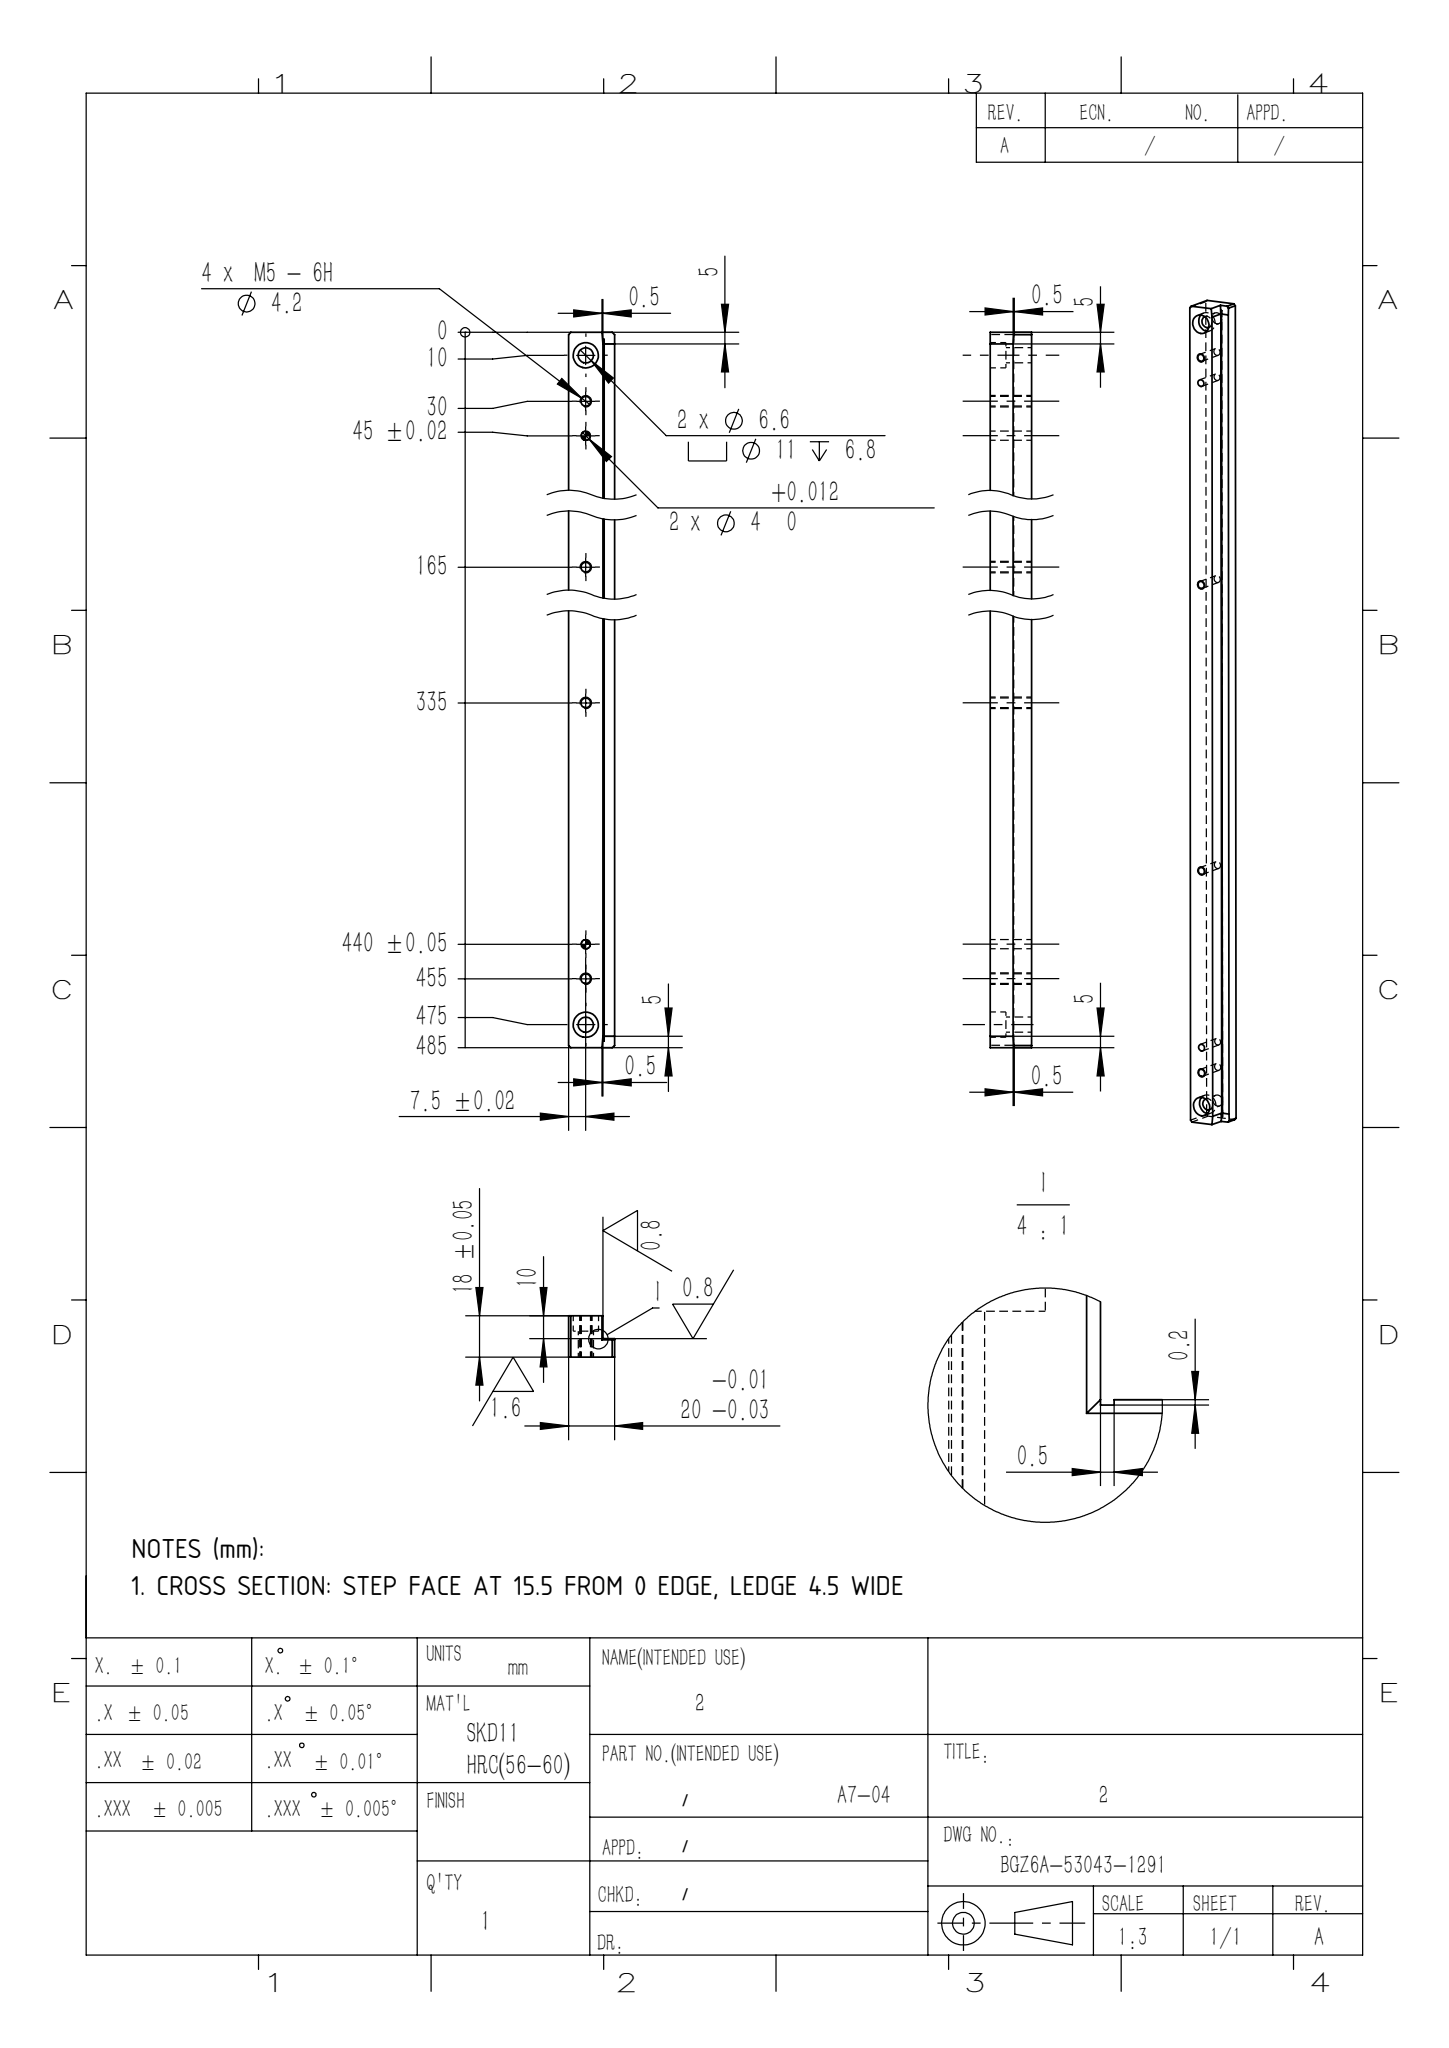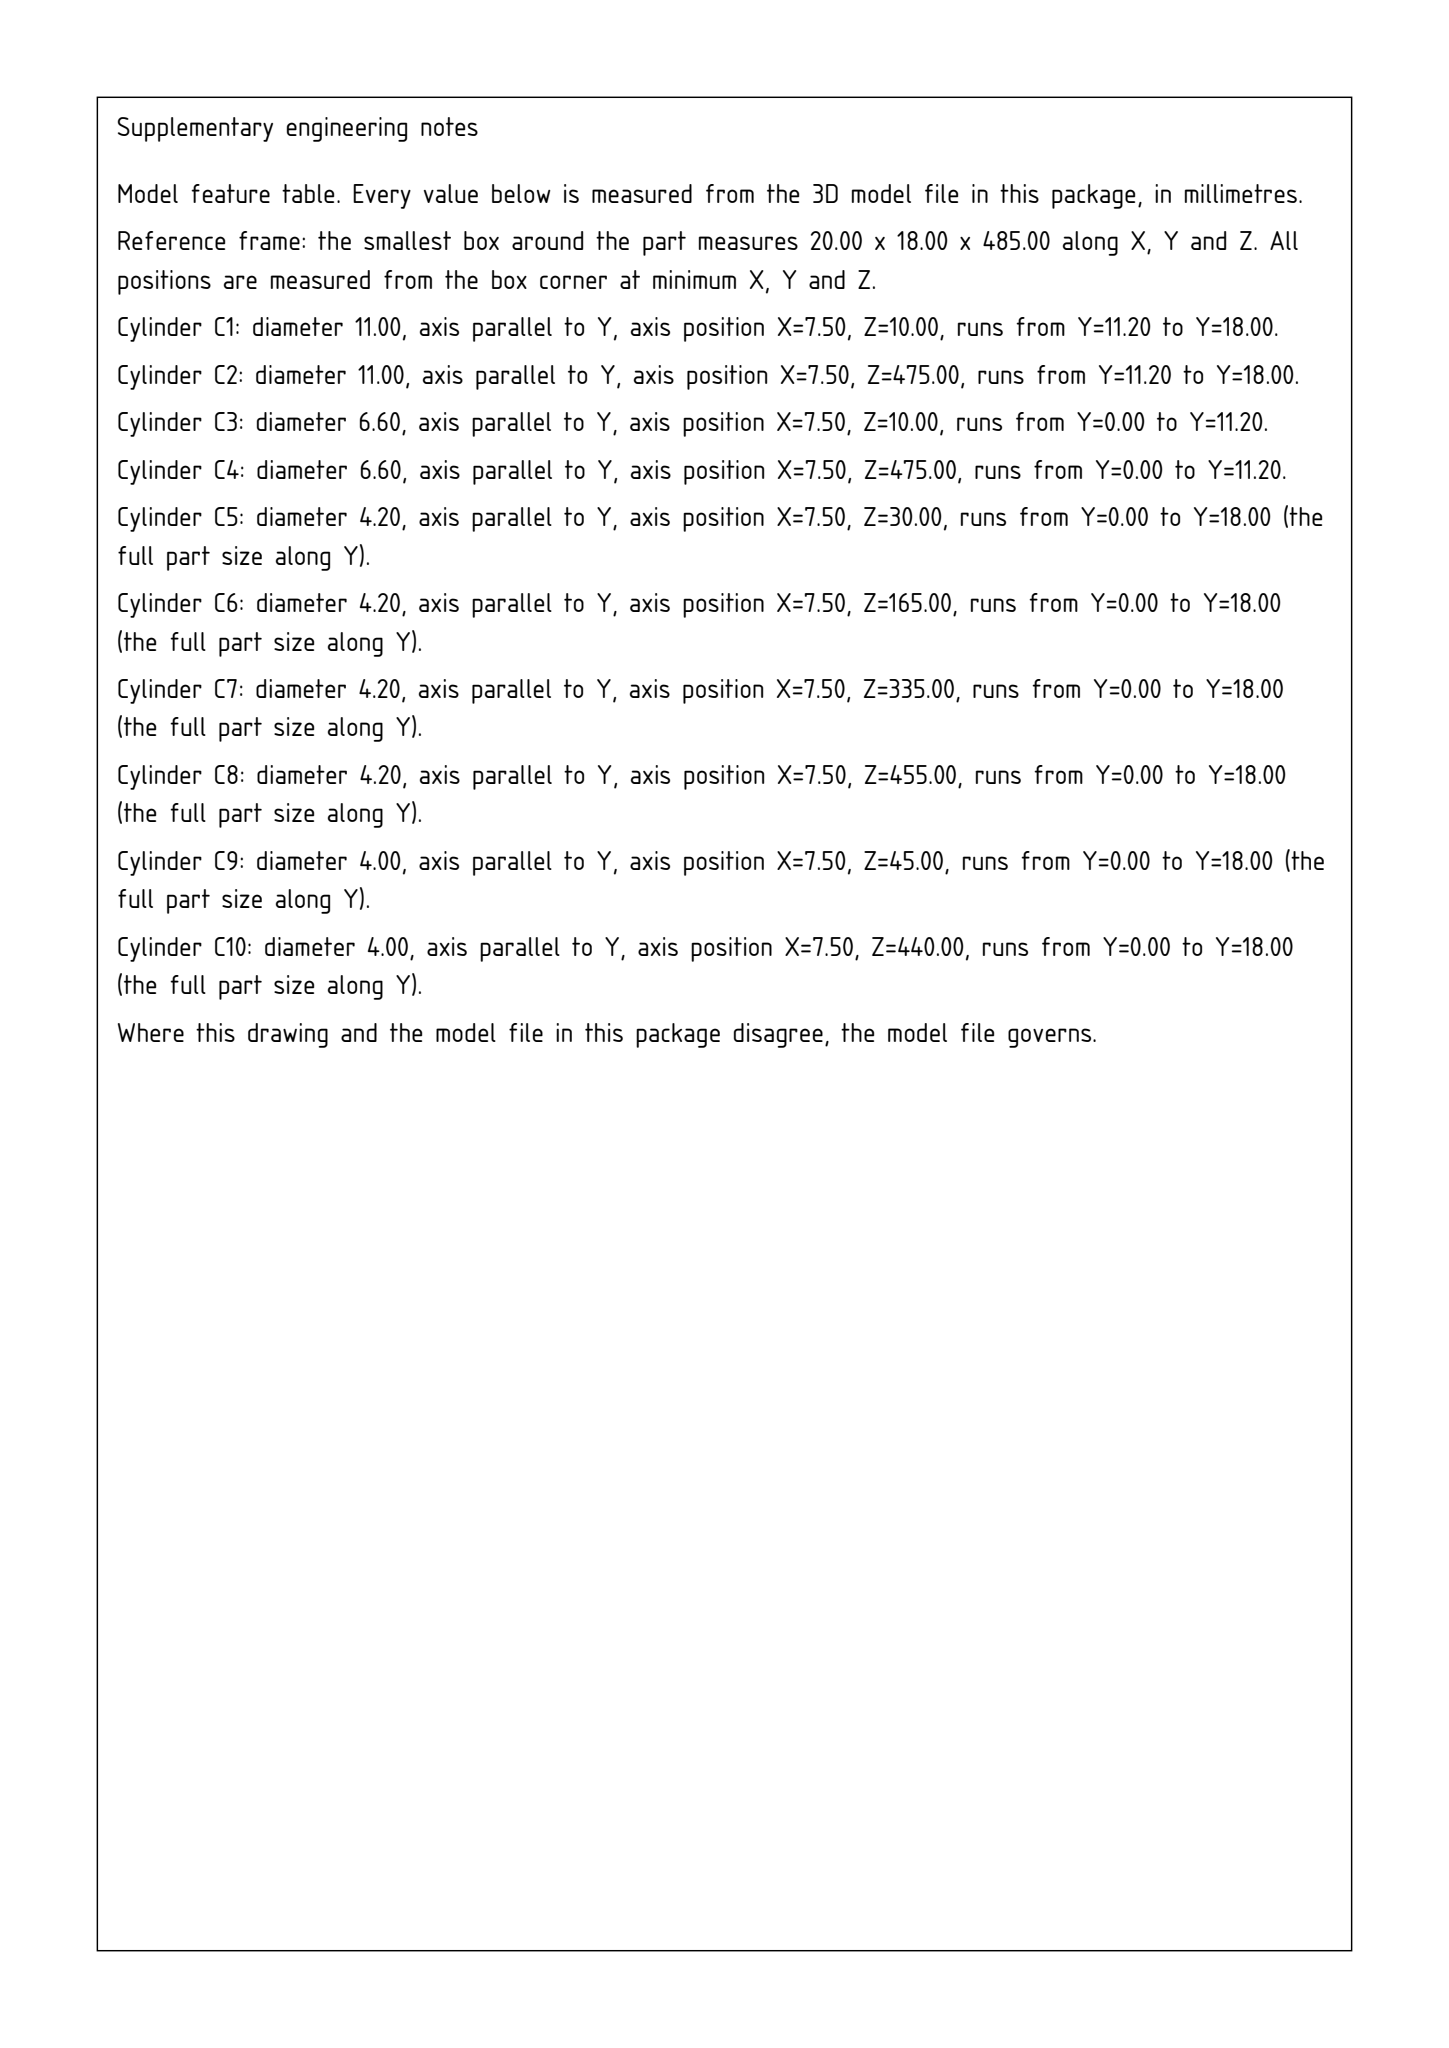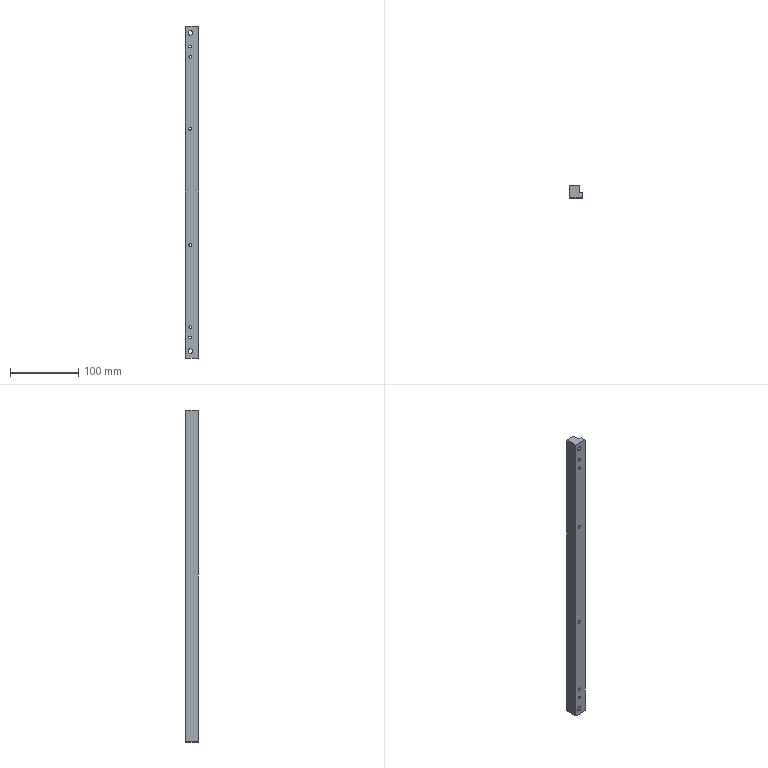Part | SolidWorks | mm | 1 solid | 40 faces | box 20 x 18 x 485 mm | volume 146730 mm3 | cylinder 20 | plane 20 | commonest cylinder face diameters 4.2 x8 4 x4 11 x4 6.6 x4
Drawing notes:
CROSS SECTION: STEP FACE AT 15.5 FROM 0 EDGE, LEDGE 4.5 WIDE | from the solid: x planes at 0, 15.0, 15.5, 20.0; 20.0-15.5 = 4.5 ledge width
build123d program:
from build123d import *
from OCP.BRepFilletAPI import BRepFilletAPI_MakeChamfer

# Parameters (mm, degrees)
BOSS_EXTRUDE1_DEPTH                             = 485
CHAMFER1_SIZE                                   = 0.5
CHAMFER1_SIZE2                                  = 5.001
SKETCH2_W                                       = 0.5
SKETCH2_H                                       = 0.2
CUT_EXTRUDE1_DEPTH                              = 486.746
M5_TAPPED_HOLE2_D                               = 4.2
M6_HEX_SOCKET_HEAD_CAP_SCREW_CBORE1_D           = 6.6
M6_HEX_SOCKET_HEAD_CAP_SCREW_CBORE1_CBORE_D     = 11
M6_HEX_SOCKET_HEAD_CAP_SCREW_CBORE1_CBORE_DEPTH = 6.8
F_4_0MM_DOWEL_PIN_HOLE_1_D                      = 4
CHAMFER2_SIZE                                   = 1


with BuildPart() as part:
    # Sketch1 → Boss-Extrude1 (new body)
    with BuildSketch(Plane.XY):
        Polygon((0, 0), (0, 18), (15, 18), (15, 8), (20, 8), (20, 0), align=None)
    extrude(amount=BOSS_EXTRUDE1_DEPTH)

    # Chamfer1: one chamfer whose edges measure the first distance from different faces: ONE call of the kernel's chamfer builder (chamfer() names one face for all edges)
    chamfer1_edges_1 = [part.edges().sort_by_distance(p)[0] for p in [
        (17.5, 8, 485),
        (15, 13, 485),
    ]]
    chamfer1_side_1 = [part.faces().sort_by_distance(p)[0] for p in [
        (8.79, 8.355, 485),
    ]]
    chamfer1_edges_2 = [part.edges().sort_by_distance(p)[0] for p in [
        (15, 13, 0),
        (17.5, 8, 0),
    ]]
    chamfer1_side_2 = [part.faces().sort_by_distance(p)[0] for p in [
        (8.79, 8.355, 0),
    ]]
    chamfer1 = BRepFilletAPI_MakeChamfer(part.part.solid().wrapped)
    for e in chamfer1_edges_1:
        chamfer1.Add(CHAMFER1_SIZE, CHAMFER1_SIZE2, e.wrapped, chamfer1_side_1[0].wrapped)  # the first distance lies on this face
    for e in chamfer1_edges_2:
        chamfer1.Add(CHAMFER1_SIZE, CHAMFER1_SIZE2, e.wrapped, chamfer1_side_2[0].wrapped)  # the first distance lies on this face
    add(Compound.cast(chamfer1.Shape()), mode=Mode.REPLACE)

    # Sketch2 → Cut-Extrude1 (cut, through all)
    with BuildSketch(Plane.XY.offset(485)):
        with Locations((15.25, 7.9)):
            Rectangle(SKETCH2_W, SKETCH2_H)
    extrude(amount=-CUT_EXTRUDE1_DEPTH, mode=Mode.SUBTRACT)

    # M5 Tapped Hole2 (through all)
    with Locations(Plane(origin=(0, 18, 0), x_dir=(1, 0, 0), z_dir=(0, 1, 0))):
        with Locations((7.5, -30), (7.5, -335), (7.5, -455), (7.5, -165)):
            Hole(M5_TAPPED_HOLE2_D / 2)

    # M6 Hex Socket Head Cap Screw CBORE1 (through all)
    with Locations(Plane(origin=(0, 18, 0), x_dir=(1, 0, 0), z_dir=(0, 1, 0))):
        with Locations((7.5, -10), (7.5, -475)):
            CounterBoreHole(M6_HEX_SOCKET_HEAD_CAP_SCREW_CBORE1_D / 2, M6_HEX_SOCKET_HEAD_CAP_SCREW_CBORE1_CBORE_D / 2, M6_HEX_SOCKET_HEAD_CAP_SCREW_CBORE1_CBORE_DEPTH)

    # 4.0mm Dowel Pin Hole 1 (through all)
    with Locations(Plane(origin=(0, 18, 0), x_dir=(1, 0, 0), z_dir=(0, 1, 0))):
        with Locations((7.5, -45), (7.5, -440)):
            Hole(F_4_0MM_DOWEL_PIN_HOLE_1_D / 2)

    # Chamfer2
    chamfer2_edges = [part.edges().sort_by_distance(p)[0] for p in [
        (0, 9, 485),
        (0, 9, 0),
        (20, 3.75, 0),
        (20, 3.75, 485),
    ]]
    chamfer(chamfer2_edges, length=CHAMFER2_SIZE)


solid = part.part